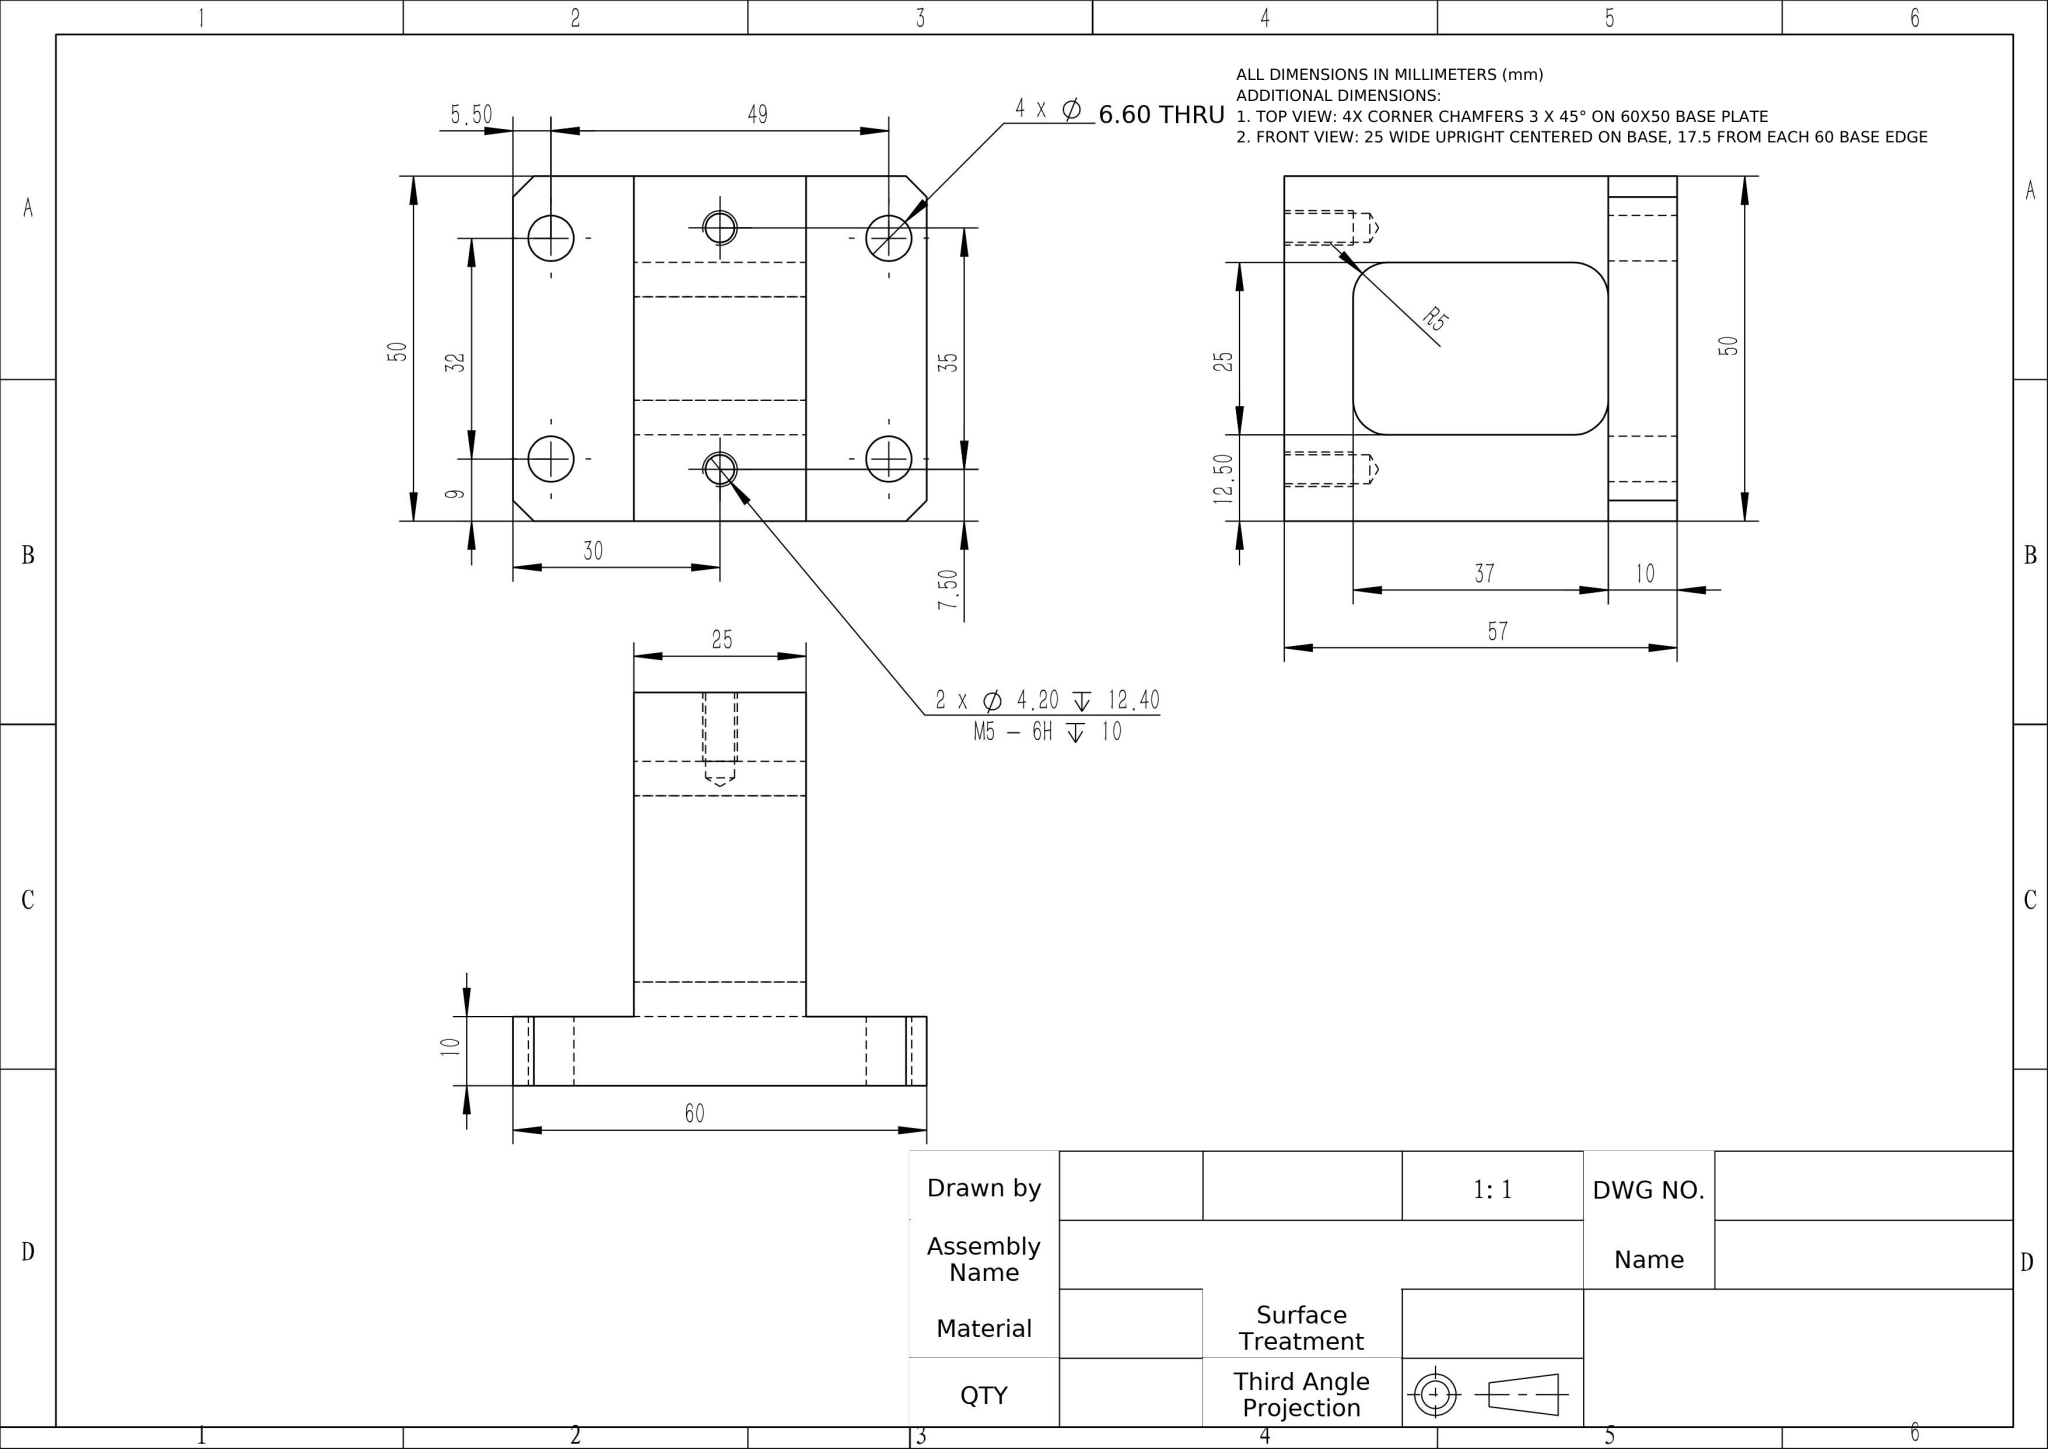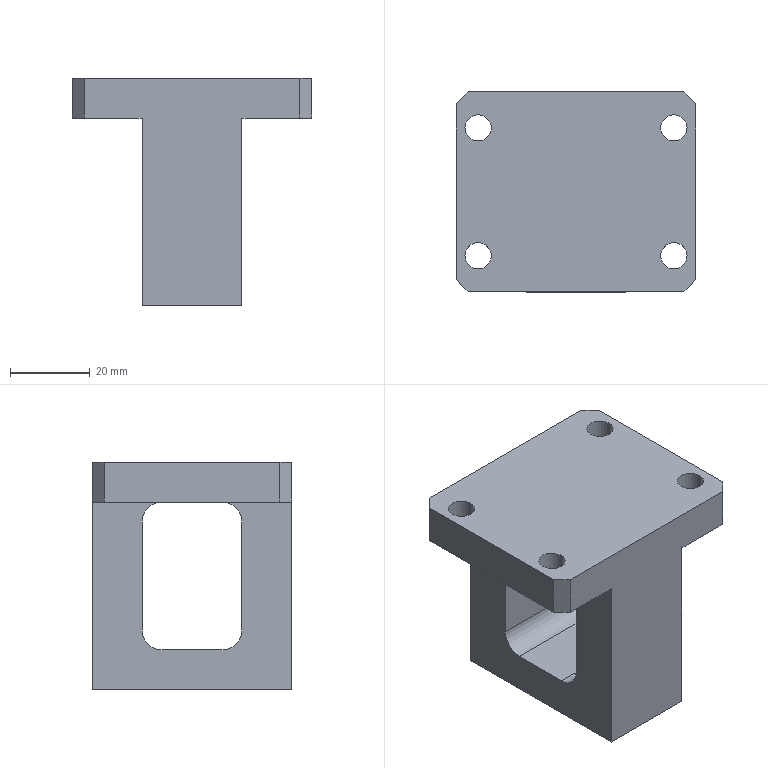Part | NX | mm | 1 solid | 36 faces | box 60 x 50 x 57 mm | volume 64258 mm3 | cylinder 16 | plane 16 | cone 4 | commonest cylinder face diameters 6.6 x8 4.2 x4 10 x4